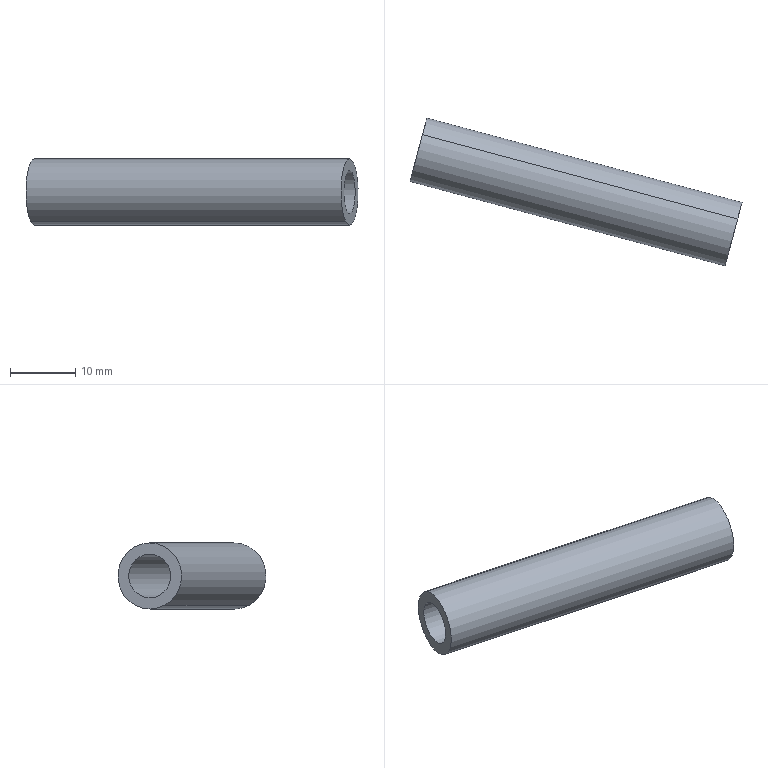Component | SolidWorks | ScrewFeedConnectorAssembly-1_AirTube-3 | 1 solid | 6 faces | box 50.92 x 22.72 x 10.12 mm | volume 2275 mm3 | cylinder 4 | plane 2 | commonest cylinder face diameters 6.67 x2 10.12 x2
build123d program:
from build123d import *

# Parameters (mm, degrees)
SKETCH1_R           = 5.06
SKETCH1_R_2         = 3.335
BOSS_EXTRUDE1_DEPTH = 50


with BuildPart() as part:
    # Sketch1 → Boss-Extrude1 (new body)
    with BuildSketch(Plane.XY):
        Circle(SKETCH1_R)
        Circle(SKETCH1_R_2, mode=Mode.SUBTRACT)
    extrude(amount=BOSS_EXTRUDE1_DEPTH)


solid = part.part

# Placed as in the assembly
solid = solid.moved(Location((-56.033, 104.137, 11), (90, 75, 107.051)))
STEP:
#1=COLOUR_RGB('',0.7922,0.8196,0.9333);
#2=FILL_AREA_STYLE_COLOUR('',#1);
#3=FILL_AREA_STYLE('',(#2));
#4=SURFACE_STYLE_FILL_AREA(#3);
#5=SURFACE_SIDE_STYLE('',(#4));
#6=SURFACE_STYLE_USAGE(.BOTH.,#5);
#7=PRESENTATION_STYLE_ASSIGNMENT((#6));
#8=CARTESIAN_POINT('',(-0.2885,3.65,0.5487));
#9=VERTEX_POINT('',#8);
#10=CARTESIAN_POINT('',(-0.3207,3.53,0.3174));
#11=VERTEX_POINT('',#10);
#12=CARTESIAN_POINT('',(-0.3046,3.59,0.4331));
#13=DIRECTION('',(0.9659,-0.2588,0.));
#14=DIRECTION('',(-0.1226,-0.4575,-0.8807));
#15=AXIS2_PLACEMENT_3D('',#12,#13,#14);
#16=CIRCLE('',#15,0.1313);
#17=EDGE_CURVE('',#9,#11,#16,.T.);
#18=ORIENTED_EDGE('',*,*,#17,.T.);
#19=CARTESIAN_POINT('',(-2.222,4.04,0.3174));
#20=VERTEX_POINT('',#19);
#21=CARTESIAN_POINT('',(-0.3207,3.53,0.3174));
#22=DIRECTION('',(-0.9659,0.2588,-0.));
#23=VECTOR('',#22,39.37);
#24=LINE('',#21,#23);
#25=EDGE_CURVE('',#11,#20,#24,.T.);
#26=ORIENTED_EDGE('',*,*,#25,.T.);
#27=CARTESIAN_POINT('',(-2.19,4.16,0.5487));
#28=VERTEX_POINT('',#27);
#29=CARTESIAN_POINT('',(-2.206,4.1,0.4331));
#30=DIRECTION('',(0.9659,-0.2588,0.));
#31=DIRECTION('',(-0.1226,-0.4575,-0.8807));
#32=AXIS2_PLACEMENT_3D('',#29,#30,#31);
#33=CIRCLE('',#32,0.1313);
#34=EDGE_CURVE('',#28,#20,#33,.T.);
#35=ORIENTED_EDGE('',*,*,#34,.F.);
#36=CARTESIAN_POINT('',(-0.2885,3.65,0.5487));
#37=DIRECTION('',(-0.9659,0.2588,-0.));
#38=VECTOR('',#37,39.37);
#39=LINE('',#36,#38);
#40=EDGE_CURVE('',#9,#28,#39,.T.);
#41=ORIENTED_EDGE('',*,*,#40,.F.);
#42=EDGE_LOOP('',(#18,#26,#35,#41));
#43=FACE_OUTER_BOUND('',#42,.T.);
#44=CARTESIAN_POINT('',(-0.3046,3.59,0.4331));
#45=DIRECTION('',(-0.9659,0.2588,-0.));
#46=DIRECTION('',(0.1226,0.4575,0.8807));
#47=AXIS2_PLACEMENT_3D('',#44,#45,#46);
#48=CYLINDRICAL_SURFACE('',#47,0.1313);
#49=ADVANCED_FACE('',(#43),#48,.F.);
#50=CARTESIAN_POINT('',(-0.329,3.499,0.2576));
#51=VERTEX_POINT('',#50);
#52=CARTESIAN_POINT('',(-0.2802,3.682,0.6085));
#53=VERTEX_POINT('',#52);
#54=CARTESIAN_POINT('',(-0.3046,3.59,0.4331));
#55=DIRECTION('',(0.9659,-0.2588,0.));
#56=DIRECTION('',(-0.1226,-0.4575,-0.8807));
#57=AXIS2_PLACEMENT_3D('',#54,#55,#56);
#58=CIRCLE('',#57,0.1992);
#59=EDGE_CURVE('',#51,#53,#58,.T.);
#60=ORIENTED_EDGE('',*,*,#59,.F.);
#61=CARTESIAN_POINT('',(-2.23,4.009,0.2576));
#62=VERTEX_POINT('',#61);
#63=CARTESIAN_POINT('',(-0.329,3.499,0.2576));
#64=DIRECTION('',(-0.9659,0.2588,-0.));
#65=VECTOR('',#64,39.37);
#66=LINE('',#63,#65);
#67=EDGE_CURVE('',#51,#62,#66,.T.);
#68=ORIENTED_EDGE('',*,*,#67,.T.);
#69=CARTESIAN_POINT('',(-2.182,4.191,0.6085));
#70=VERTEX_POINT('',#69);
#71=CARTESIAN_POINT('',(-2.206,4.1,0.4331));
#72=DIRECTION('',(0.9659,-0.2588,0.));
#73=DIRECTION('',(-0.1226,-0.4575,-0.8807));
#74=AXIS2_PLACEMENT_3D('',#71,#72,#73);
#75=CIRCLE('',#74,0.1992);
#76=EDGE_CURVE('',#62,#70,#75,.T.);
#77=ORIENTED_EDGE('',*,*,#76,.T.);
#78=CARTESIAN_POINT('',(-0.2802,3.682,0.6085));
#79=DIRECTION('',(-0.9659,0.2588,-0.));
#80=VECTOR('',#79,39.37);
#81=LINE('',#78,#80);
#82=EDGE_CURVE('',#53,#70,#81,.T.);
#83=ORIENTED_EDGE('',*,*,#82,.F.);
#84=EDGE_LOOP('',(#60,#68,#77,#83));
#85=FACE_OUTER_BOUND('',#84,.T.);
#86=CARTESIAN_POINT('',(-0.3046,3.59,0.4331));
#87=DIRECTION('',(-0.9659,0.2588,-0.));
#88=DIRECTION('',(0.1226,0.4575,0.8807));
#89=AXIS2_PLACEMENT_3D('',#86,#87,#88);
#90=CYLINDRICAL_SURFACE('',#89,0.1992);
#91=ADVANCED_FACE('',(#85),#90,.T.);
#92=CARTESIAN_POINT('',(-0.3046,3.59,0.4331));
#93=DIRECTION('',(0.9659,-0.2588,0.));
#94=DIRECTION('',(-0.1226,-0.4575,-0.8807));
#95=AXIS2_PLACEMENT_3D('',#92,#93,#94);
#96=CIRCLE('',#95,0.1992);
#97=EDGE_CURVE('',#53,#51,#96,.T.);
#98=ORIENTED_EDGE('',*,*,#97,.T.);
#99=ORIENTED_EDGE('',*,*,#59,.T.);
#100=EDGE_LOOP('',(#98,#99));
#101=FACE_OUTER_BOUND('',#100,.T.);
#102=ORIENTED_EDGE('',*,*,#17,.F.);
#103=CARTESIAN_POINT('',(-0.3046,3.59,0.4331));
#104=DIRECTION('',(0.9659,-0.2588,0.));
#105=DIRECTION('',(-0.1226,-0.4575,-0.8807));
#106=AXIS2_PLACEMENT_3D('',#103,#104,#105);
#107=CIRCLE('',#106,0.1313);
#108=EDGE_CURVE('',#11,#9,#107,.T.);
#109=ORIENTED_EDGE('',*,*,#108,.F.);
#110=EDGE_LOOP('',(#102,#109));
#111=FACE_BOUND('',#110,.T.);
#112=CARTESIAN_POINT('',(-0.3046,3.59,0.4331));
#113=DIRECTION('',(0.9659,-0.2588,0.));
#114=DIRECTION('',(-0.1226,-0.4575,-0.8807));
#115=AXIS2_PLACEMENT_3D('',#112,#113,#114);
#116=PLANE('',#115);
#117=ADVANCED_FACE('',(#101,#111),#116,.T.);
#118=CARTESIAN_POINT('',(-2.206,4.1,0.4331));
#119=DIRECTION('',(0.9659,-0.2588,0.));
#120=DIRECTION('',(-0.1226,-0.4575,-0.8807));
#121=AXIS2_PLACEMENT_3D('',#118,#119,#120);
#122=CIRCLE('',#121,0.1992);
#123=EDGE_CURVE('',#70,#62,#122,.T.);
#124=ORIENTED_EDGE('',*,*,#123,.F.);
#125=ORIENTED_EDGE('',*,*,#76,.F.);
#126=EDGE_LOOP('',(#124,#125));
#127=FACE_OUTER_BOUND('',#126,.T.);
#128=ORIENTED_EDGE('',*,*,#34,.T.);
#129=CARTESIAN_POINT('',(-2.206,4.1,0.4331));
#130=DIRECTION('',(0.9659,-0.2588,0.));
#131=DIRECTION('',(-0.1226,-0.4575,-0.8807));
#132=AXIS2_PLACEMENT_3D('',#129,#130,#131);
#133=CIRCLE('',#132,0.1313);
#134=EDGE_CURVE('',#20,#28,#133,.T.);
#135=ORIENTED_EDGE('',*,*,#134,.T.);
#136=EDGE_LOOP('',(#128,#135));
#137=FACE_BOUND('',#136,.T.);
#138=CARTESIAN_POINT('',(-2.206,4.1,0.4331));
#139=DIRECTION('',(0.9659,-0.2588,0.));
#140=DIRECTION('',(-0.1226,-0.4575,-0.8807));
#141=AXIS2_PLACEMENT_3D('',#138,#139,#140);
#142=PLANE('',#141);
#143=ADVANCED_FACE('',(#127,#137),#142,.F.);
#144=ORIENTED_EDGE('',*,*,#67,.F.);
#145=ORIENTED_EDGE('',*,*,#97,.F.);
#146=ORIENTED_EDGE('',*,*,#82,.T.);
#147=ORIENTED_EDGE('',*,*,#123,.T.);
#148=EDGE_LOOP('',(#144,#145,#146,#147));
#149=FACE_OUTER_BOUND('',#148,.T.);
#150=CARTESIAN_POINT('',(-0.3046,3.59,0.4331));
#151=DIRECTION('',(-0.9659,0.2588,-0.));
#152=DIRECTION('',(0.1226,0.4575,0.8807));
#153=AXIS2_PLACEMENT_3D('',#150,#151,#152);
#154=CYLINDRICAL_SURFACE('',#153,0.1992);
#155=ADVANCED_FACE('',(#149),#154,.T.);
#156=ORIENTED_EDGE('',*,*,#25,.F.);
#157=ORIENTED_EDGE('',*,*,#108,.T.);
#158=ORIENTED_EDGE('',*,*,#40,.T.);
#159=ORIENTED_EDGE('',*,*,#134,.F.);
#160=EDGE_LOOP('',(#156,#157,#158,#159));
#161=FACE_OUTER_BOUND('',#160,.T.);
#162=CARTESIAN_POINT('',(-0.3046,3.59,0.4331));
#163=DIRECTION('',(-0.9659,0.2588,-0.));
#164=DIRECTION('',(0.1226,0.4575,0.8807));
#165=AXIS2_PLACEMENT_3D('',#162,#163,#164);
#166=CYLINDRICAL_SURFACE('',#165,0.1313);
#167=ADVANCED_FACE('',(#161),#166,.F.);
#168=CLOSED_SHELL('',(#49,#91,#117,#143,#155,#167));
#169=MANIFOLD_SOLID_BREP('',#168);
#170=STYLED_ITEM('',(#7),#169);
#171=(LENGTH_UNIT()NAMED_UNIT(*)SI_UNIT($,.METRE.));
#172=LENGTH_MEASURE_WITH_UNIT(LENGTH_MEASURE(0.0254),#171);
#173=DIMENSIONAL_EXPONENTS(1.,0.,0.,0.,0.,0.,0.);
#174=(CONVERSION_BASED_UNIT('',#172)LENGTH_UNIT()NAMED_UNIT(#173));
#175=UNCERTAINTY_MEASURE_WITH_UNIT(LENGTH_MEASURE(0.00001),#174,'','');
#176=(NAMED_UNIT(*)PLANE_ANGLE_UNIT()SI_UNIT($,.RADIAN.));
#177=(NAMED_UNIT(*)SI_UNIT($,.STERADIAN.)SOLID_ANGLE_UNIT());
#178=(GEOMETRIC_REPRESENTATION_CONTEXT(3)GLOBAL_UNCERTAINTY_ASSIGNED_CONTEXT((#175))GLOBAL_UNIT_ASSIGNED_CONTEXT((#174,#176,#177))REPRESENTATION_CONTEXT('',''));
#179=MECHANICAL_DESIGN_GEOMETRIC_PRESENTATION_REPRESENTATION('',(#170),#178);
#180=CARTESIAN_POINT('',(0.,0.,0.));
#181=DIRECTION('',(0.,0.,1.));
#182=DIRECTION('',(1.,0.,0.));
#183=AXIS2_PLACEMENT_3D('',#180,#181,#182);
#184=(LENGTH_UNIT()NAMED_UNIT(*)SI_UNIT($,.METRE.));
#185=LENGTH_MEASURE_WITH_UNIT(LENGTH_MEASURE(0.0254),#184);
#186=DIMENSIONAL_EXPONENTS(1.,0.,0.,0.,0.,0.,0.);
#187=(CONVERSION_BASED_UNIT('',#185)LENGTH_UNIT()NAMED_UNIT(#186));
#188=UNCERTAINTY_MEASURE_WITH_UNIT(LENGTH_MEASURE(0.00001),#187,'','');
#189=(NAMED_UNIT(*)PLANE_ANGLE_UNIT()SI_UNIT($,.RADIAN.));
#190=(NAMED_UNIT(*)SI_UNIT($,.STERADIAN.)SOLID_ANGLE_UNIT());
#191=(GEOMETRIC_REPRESENTATION_CONTEXT(3)GLOBAL_UNCERTAINTY_ASSIGNED_CONTEXT((#188))GLOBAL_UNIT_ASSIGNED_CONTEXT((#187,#189,#190))REPRESENTATION_CONTEXT('',''));
#192=ADVANCED_BREP_SHAPE_REPRESENTATION('',(#169,#183),#191);
#193=PRESENTATION_LAYER_ASSIGNMENT('','',(#170));